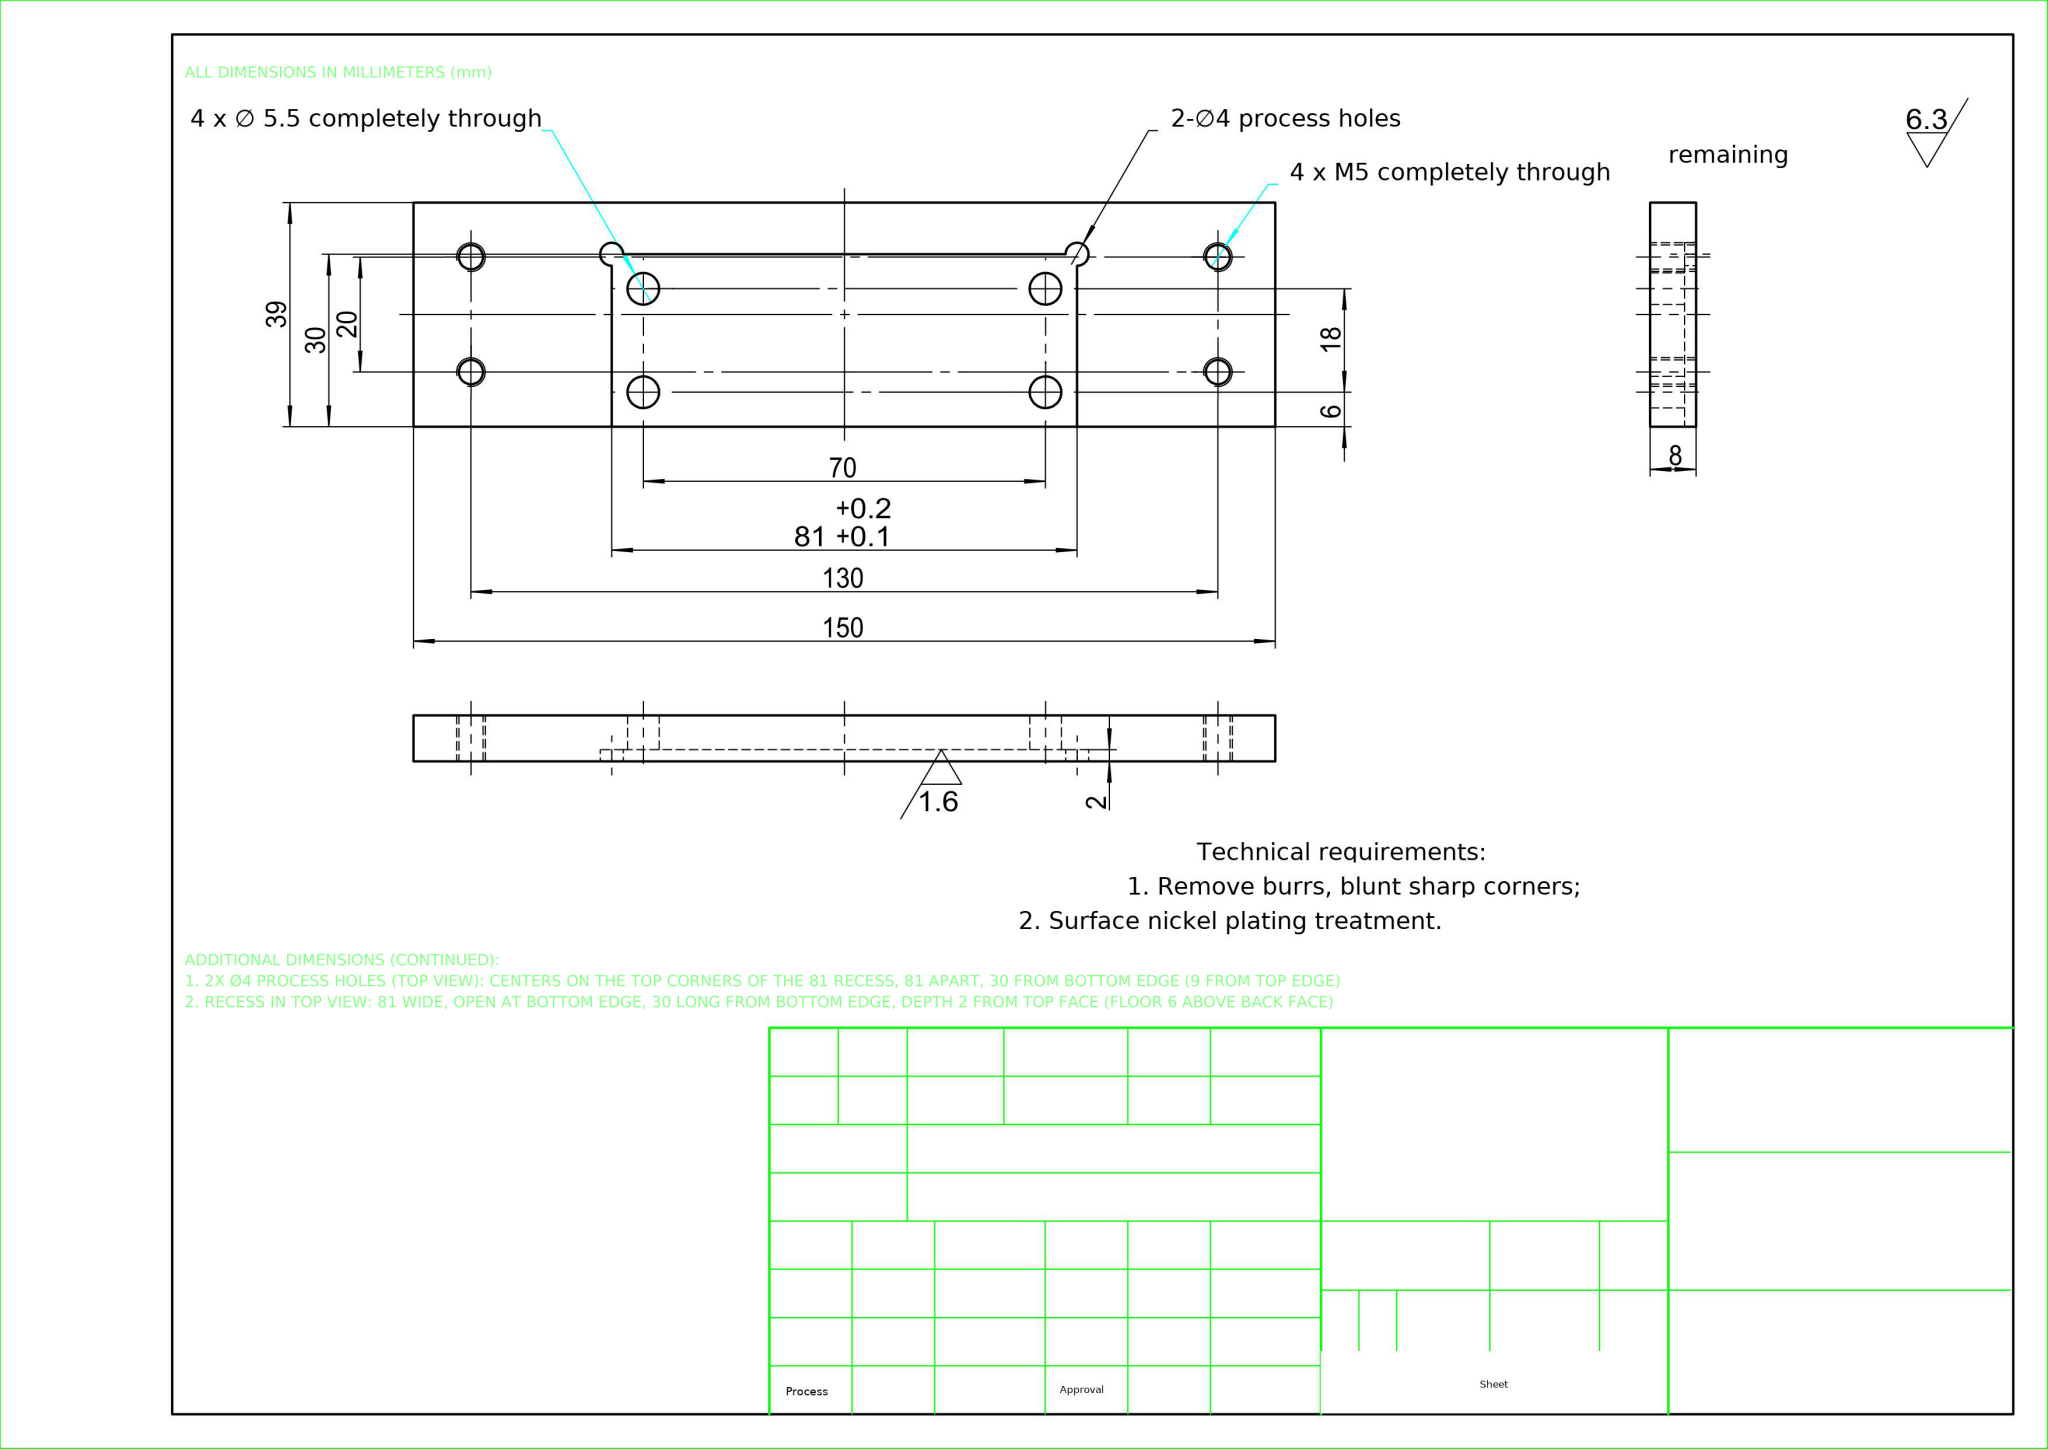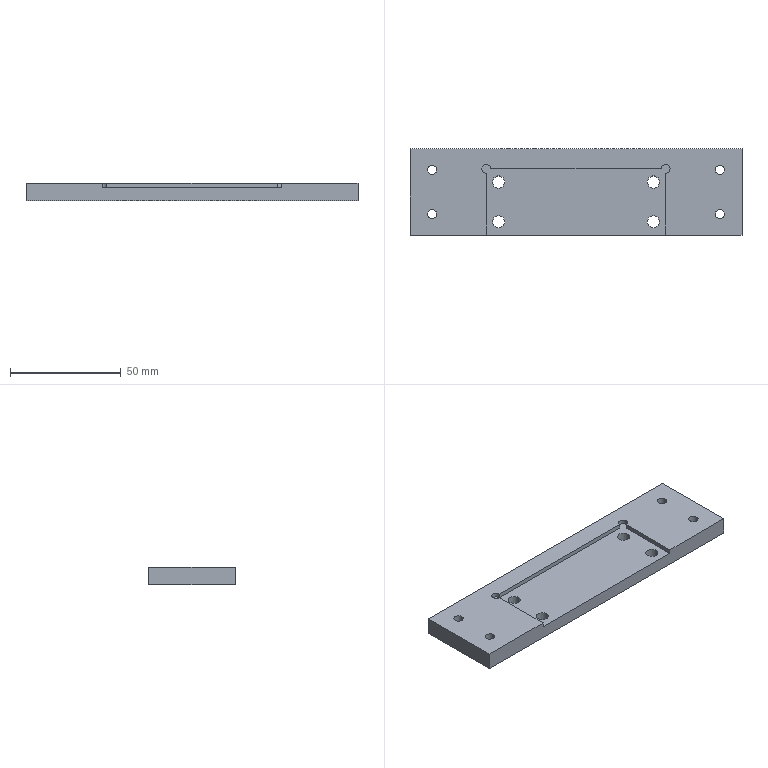Part | NX | mm | 1 solid | 29 faces | box 150 x 39 x 8 mm | volume 40889 mm3 | cylinder 19 | plane 10 | commonest cylinder face diameters 4.2 x8 5.5 x8 4 x3